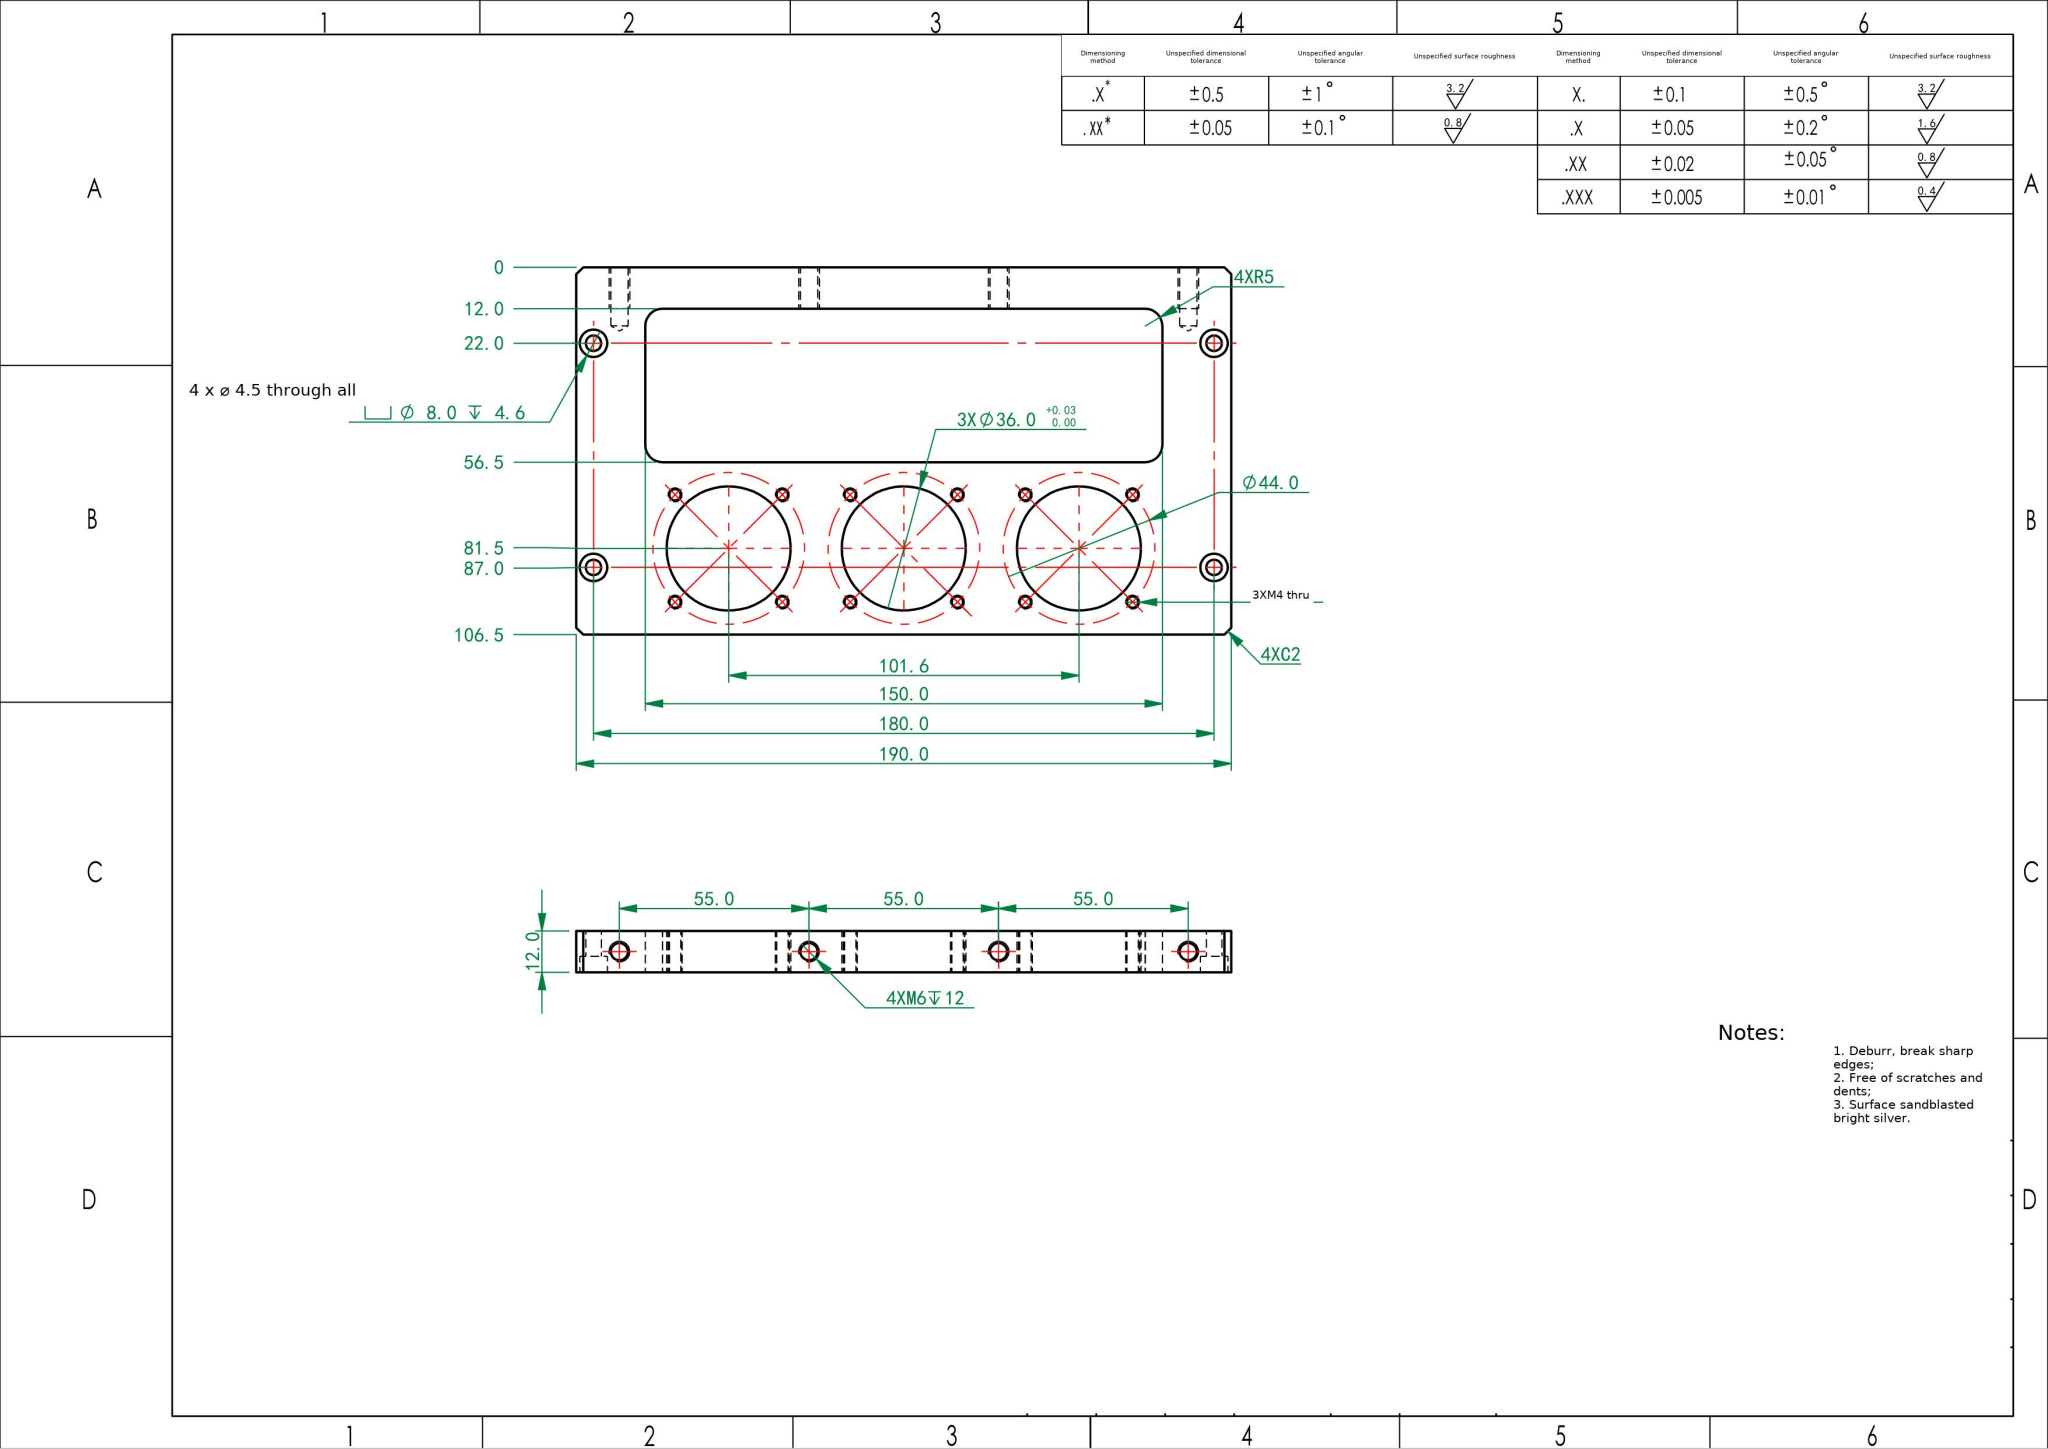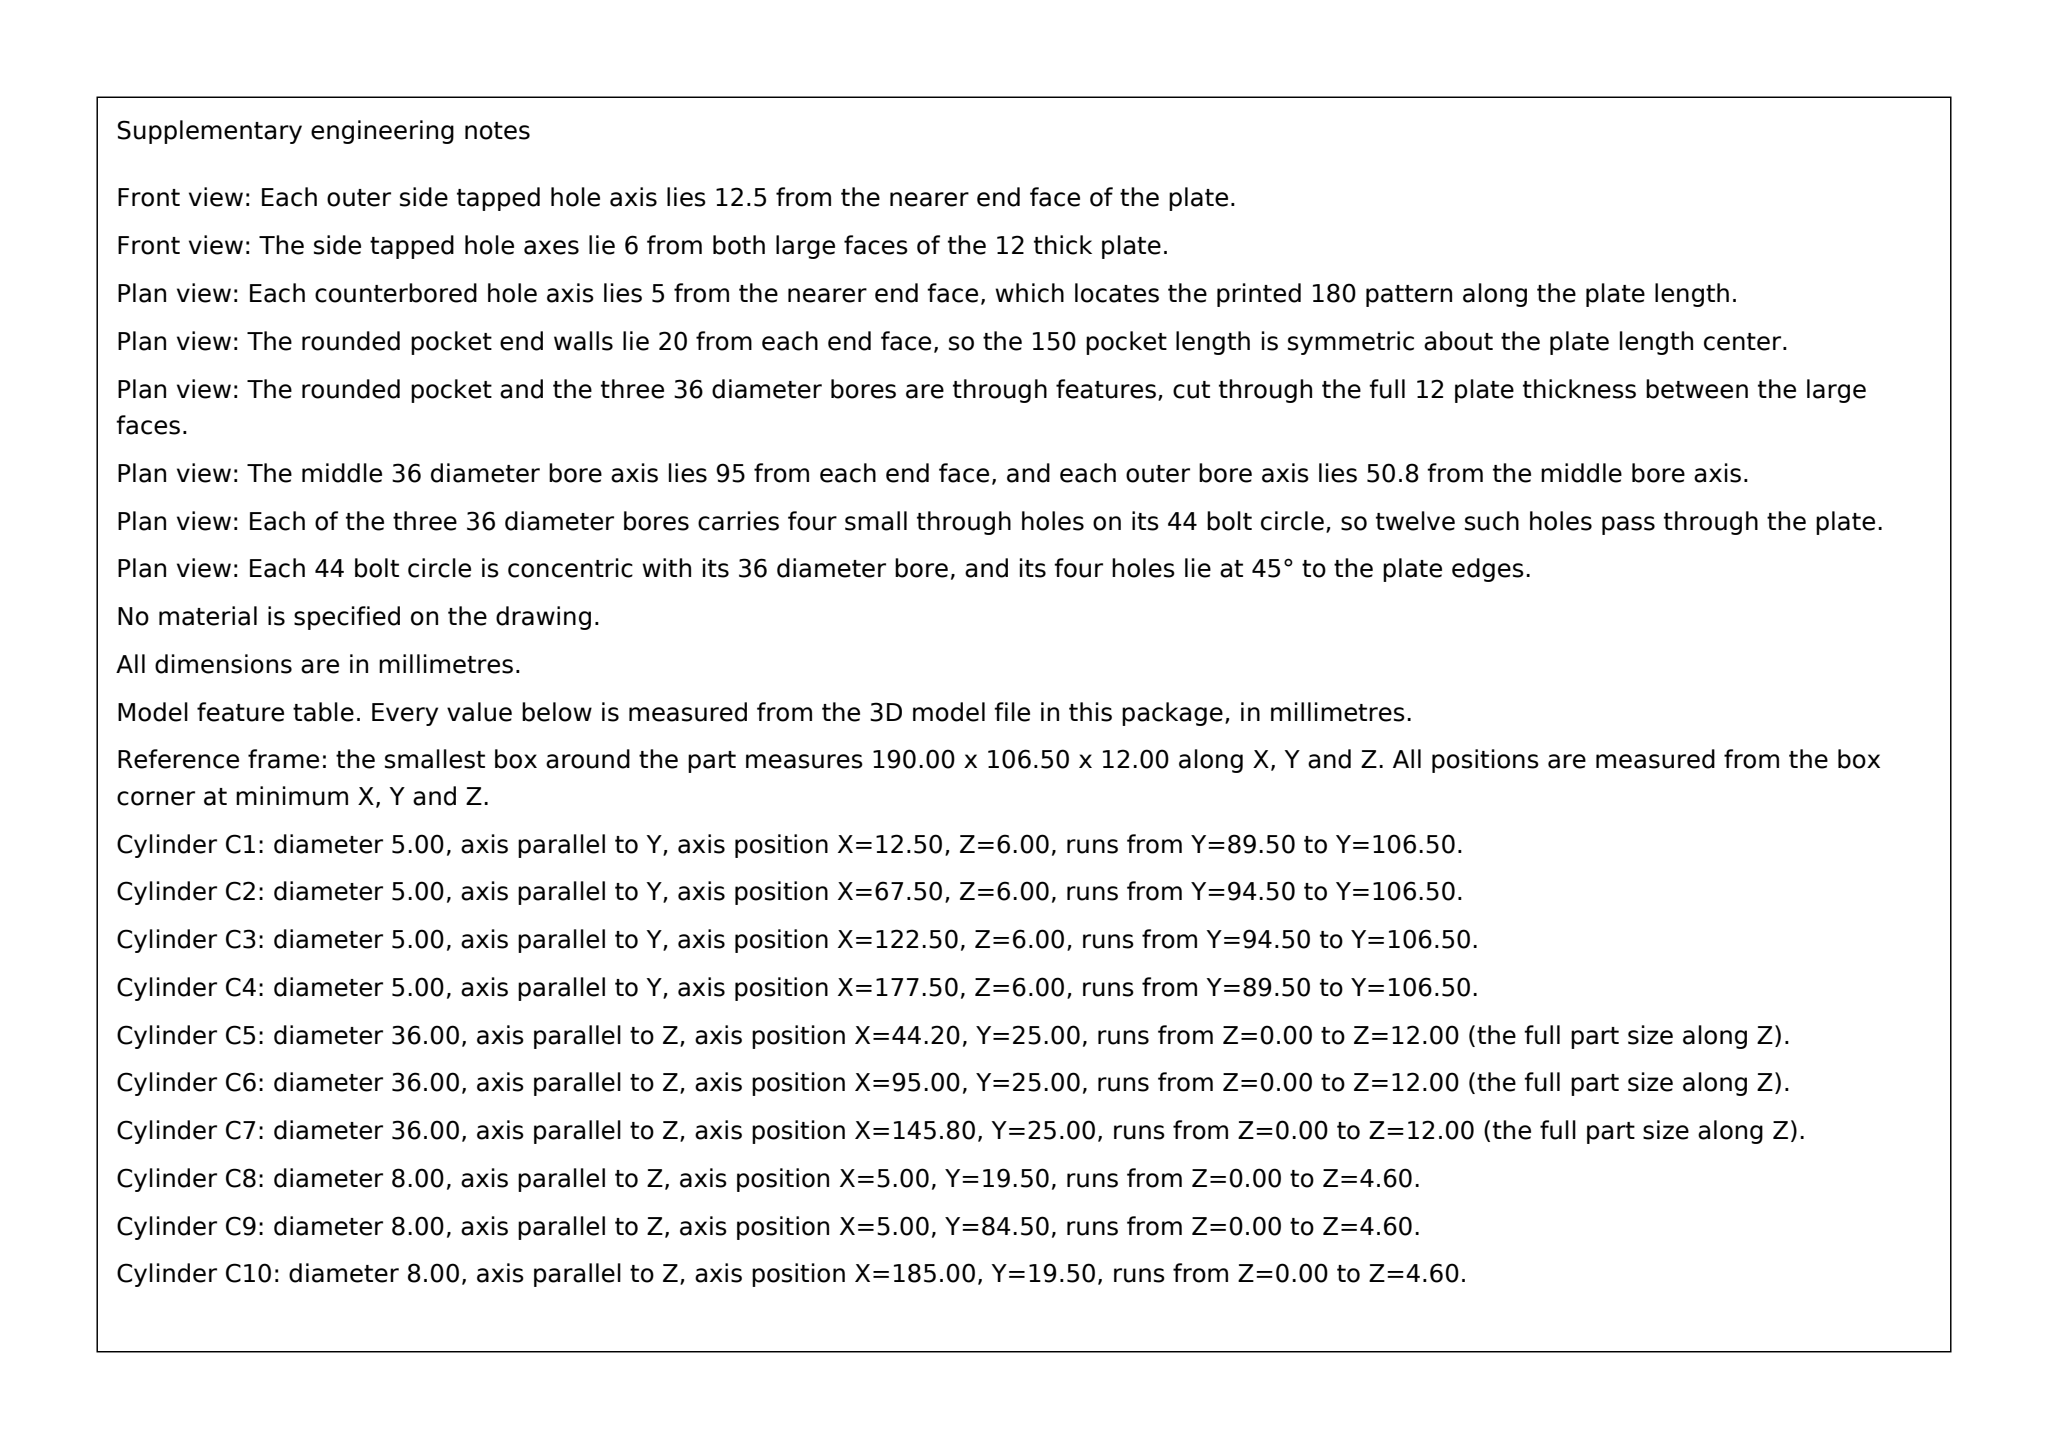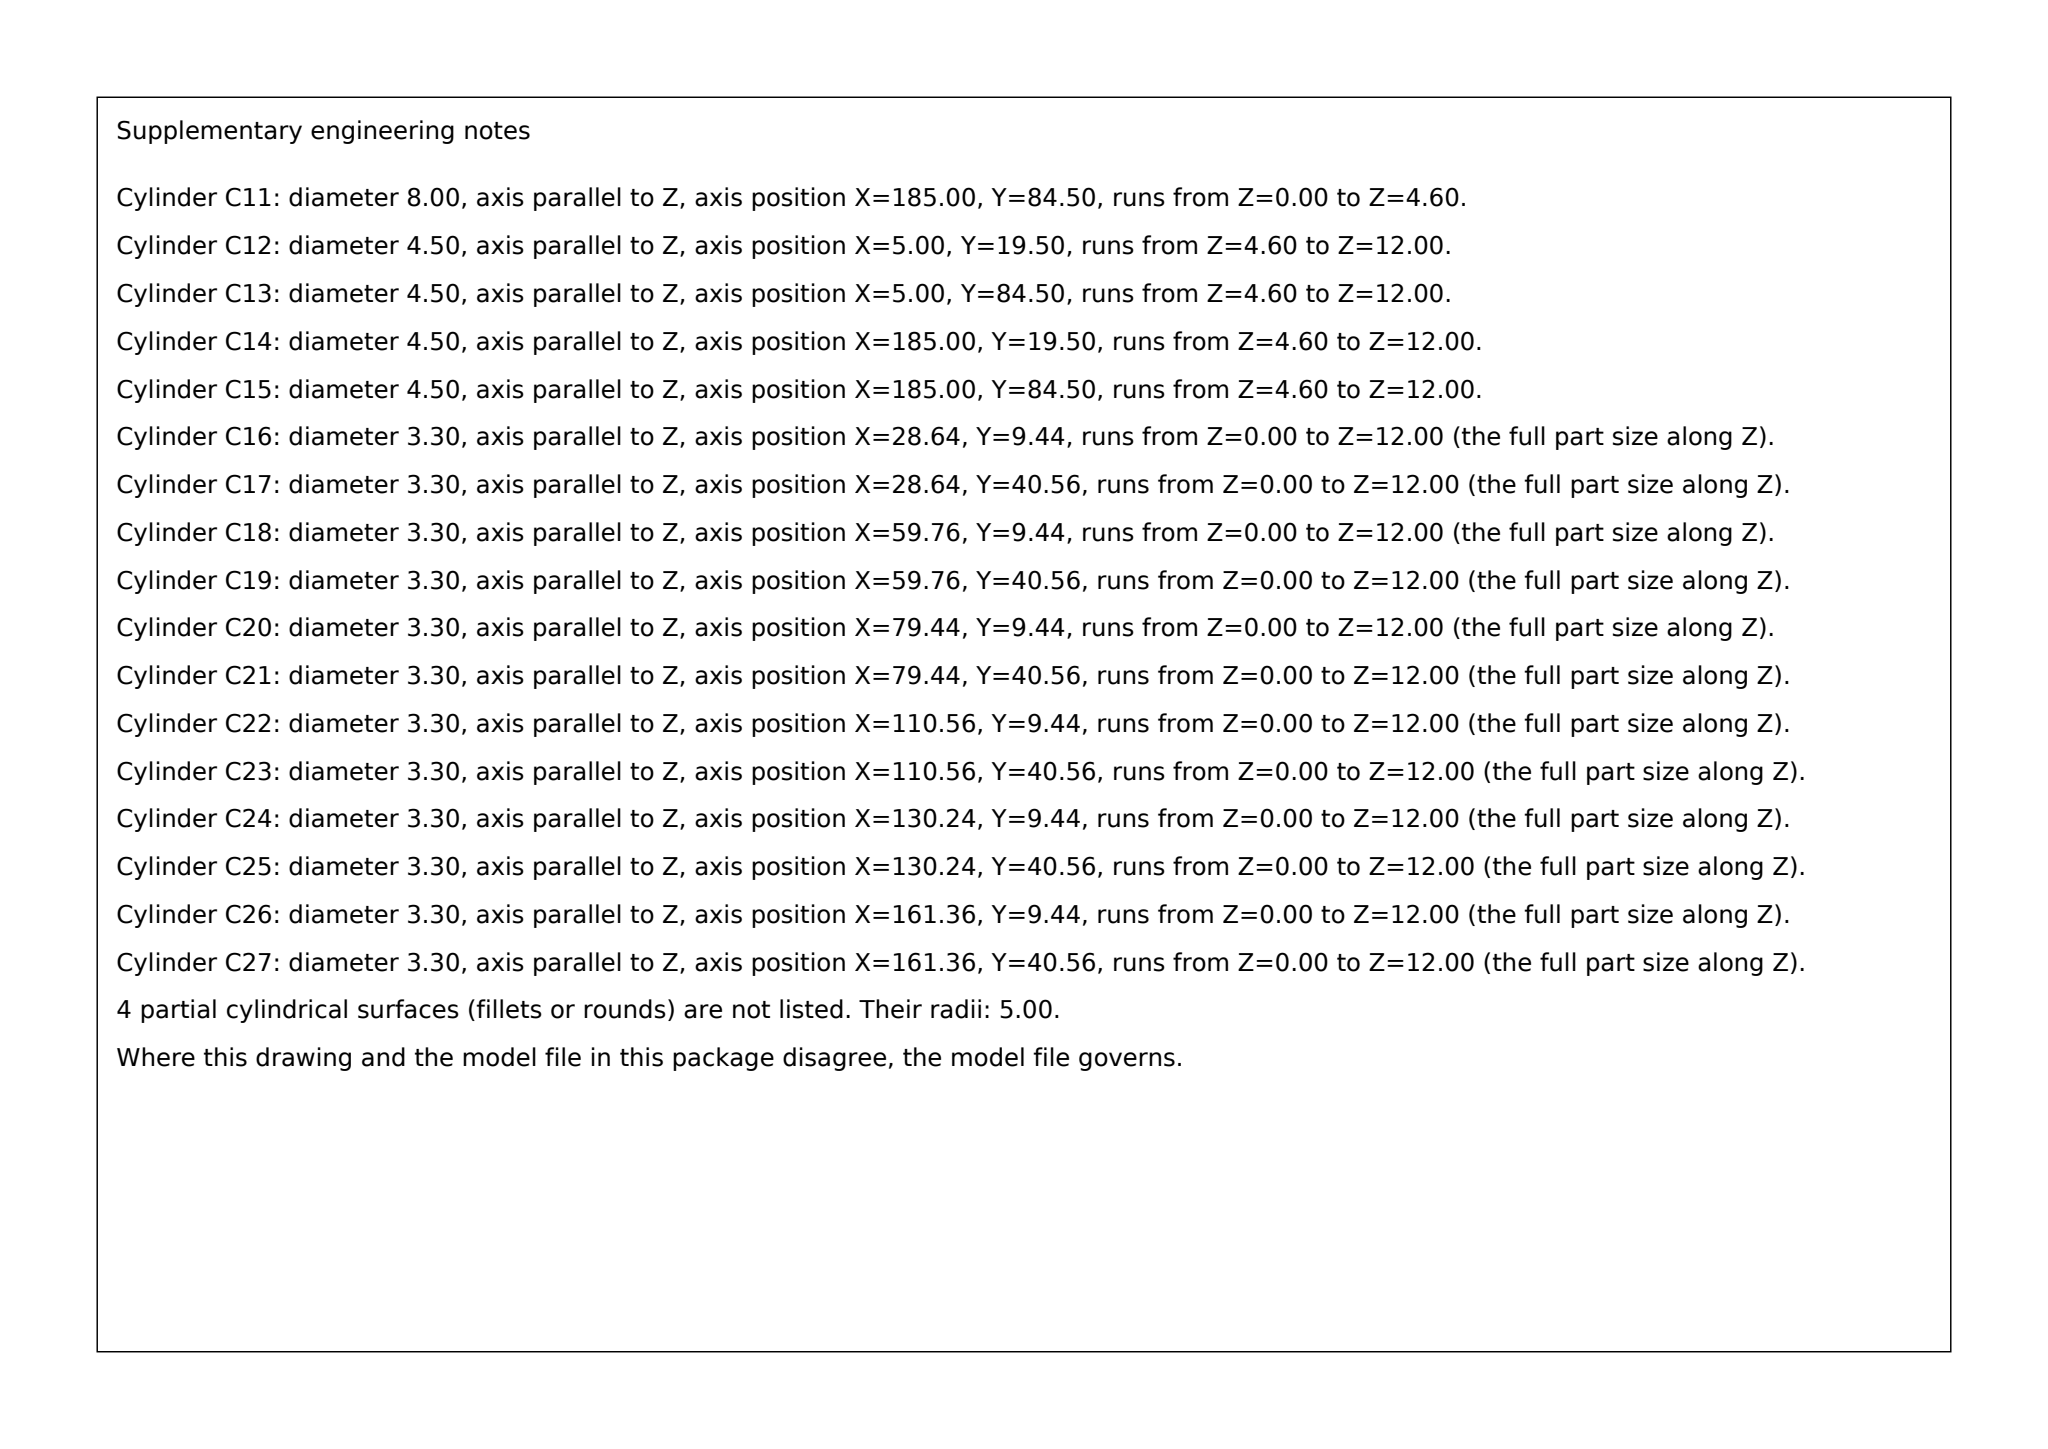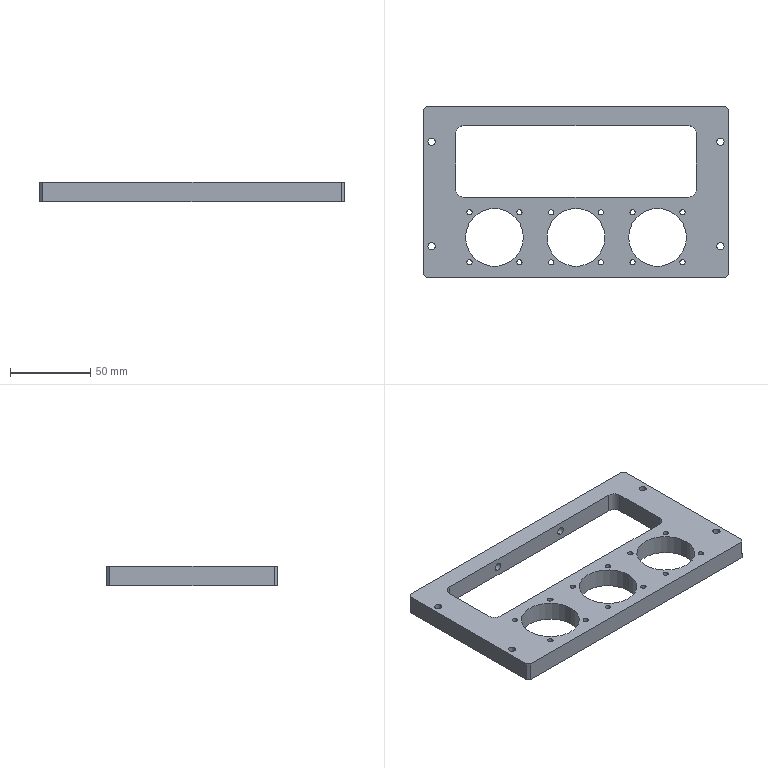Part | SolidWorks | mm | 1 solid | 80 faces | box 190 x 106.5 x 12 mm | volume 122452 mm3 | cylinder 58 | plane 18 | cone 4 | commonest cylinder face diameters 3.3 x24 8 x8 4.5 x8 5 x8 36 x6 10 x4
Drawing notes:
12X M4 THRU: 4X EA BORE, EQ SP ON Ø44.0 B.C. AT 45° TO C/L | from the solid: 24 Ø3.3 z-cylinders (12 thru, L=12.0) at ±15.56,±15.56 from each Ø36.0 bore center (44.2,25 / 95.0,25 / 145.8,25) = R22.0 at 45°
Ø44.0 B.C. TYP 3X Ø36.0 BORES | from the solid: Identical 15.56/15.56 hole pattern (R22.0) repeats about all three Ø36.0 bores at x=44.2, 95.0, 145.8
build123d program:
from build123d import *

# Parameters (mm, degrees)
SKETCH1_W                                         = 190
SKETCH1_H                                         = 106.5
BOSS_EXTRUDE1_DEPTH                               = 12
SKETCH2_R                                         = 18
CUT_EXTRUDE1_DEPTH                                = 35
M4_TAPPED_HOLE1_D                                 = 3.3
LPATTERN1_COUNT                                   = 3
LPATTERN1_PITCH                                   = 50.8
M6_TAPPED_HOLE1_D                                 = 5
M6_TAPPED_HOLE1_DEPTH                             = 17
M6_TAPPED_HOLE1_TIP                               = 1.502
HOLE_SIZE_ACCORDING_TO_HEXAGON_SOCKET_D           = 4.5
HOLE_SIZE_ACCORDING_TO_HEXAGON_SOCKET_CBORE_D     = 8
HOLE_SIZE_ACCORDING_TO_HEXAGON_SOCKET_CBORE_DEPTH = 4.6
CUT_EXTRUDE2_DEPTH                                = 84
CHAMFER1_SIZE                                     = 2


with BuildPart() as part:
    # Sketch1 → Boss-Extrude1 (new body)
    with BuildSketch(Plane.XY):
        Rectangle(SKETCH1_W, SKETCH1_H)
    extrude(amount=BOSS_EXTRUDE1_DEPTH)

    # Sketch2 → Cut-Extrude1 (cut)
    with BuildSketch(Plane.XY.offset(12)):
        with Locations((0, -28.25)):
            Circle(SKETCH2_R)
        with Locations((-50.8, -28.25)):
            Circle(SKETCH2_R)
        with Locations((50.8, -28.25)):
            Circle(SKETCH2_R)
    extrude(amount=-CUT_EXTRUDE1_DEPTH, mode=Mode.SUBTRACT)

    # M4 Tapped Hole1 (through all)
    with Locations(Plane(origin=(-66.356, -12.694, 12), x_dir=(1, 0, 0), z_dir=(0, 0, 1))):
        with Locations((0, 0), (31.113, 0), (31.113, -31.113), (0, -31.113)):
            m4_tapped_hole1 = Hole(M4_TAPPED_HOLE1_D / 2)

    # LPattern1: M4 Tapped Hole1 ×3
    with Locations(*[(i * LPATTERN1_PITCH, 0, 0) for i in range(1, LPATTERN1_COUNT)]):
        add(m4_tapped_hole1, mode=Mode.SUBTRACT)

    # M6 Tapped Hole1
    with Locations(Plane(origin=(-82.5, 53.25, 6), x_dir=(0, 0, 1), z_dir=(0, 1, 0))):
        with Locations((0, 0), (0, 55), (0, 110), (0, 165)):
            Hole(M6_TAPPED_HOLE1_D / 2, depth=M6_TAPPED_HOLE1_DEPTH)
            with Locations((0, 0, -(M6_TAPPED_HOLE1_DEPTH + M6_TAPPED_HOLE1_TIP / 2))):  # 118° drill point
                Cone(0, M6_TAPPED_HOLE1_D / 2, M6_TAPPED_HOLE1_TIP, mode=Mode.SUBTRACT)

    # Hole Size _ according to_ Hexagon Socket (through all)
    with Locations(Plane(origin=(-90, 31.25, 0), x_dir=(-1, 0, 0), z_dir=(0, 0, -1))):
        with Locations((0, 0), (0, -65), (-180, -65), (-180, 0)):
            CounterBoreHole(HOLE_SIZE_ACCORDING_TO_HEXAGON_SOCKET_D / 2, HOLE_SIZE_ACCORDING_TO_HEXAGON_SOCKET_CBORE_D / 2, HOLE_SIZE_ACCORDING_TO_HEXAGON_SOCKET_CBORE_DEPTH)

    # Sketch9 → Cut-Extrude2 (cut)
    with BuildSketch(Plane(origin=(0, 0, 0), x_dir=(-1, 0, 0), z_dir=(0, 0, -1))):
        with BuildLine():
            Line((-70, 41.25), (70, 41.25))
            ThreePointArc((70, 41.25), (73.536, 39.786), (75, 36.25))
            Line((75, 36.25), (75, 1.75))
            ThreePointArc((75, 1.75), (73.536, -1.786), (70, -3.25))
            Line((70, -3.25), (-70, -3.25))
            ThreePointArc((-70, -3.25), (-73.536, -1.786), (-75, 1.75))
            Line((-75, 1.75), (-75, 36.25))
            ThreePointArc((-75, 36.25), (-73.536, 39.786), (-70, 41.25))
        make_face()
    extrude(amount=-CUT_EXTRUDE2_DEPTH, mode=Mode.SUBTRACT)

    # Chamfer1
    chamfer1_edges = [part.edges().sort_by_distance(p)[0] for p in [
        (95, -53.25, 6),
        (-95, -53.25, 6),
        (-95, 53.25, 6),
        (95, 53.25, 6),
    ]]
    chamfer(chamfer1_edges, length=CHAMFER1_SIZE)


solid = part.part